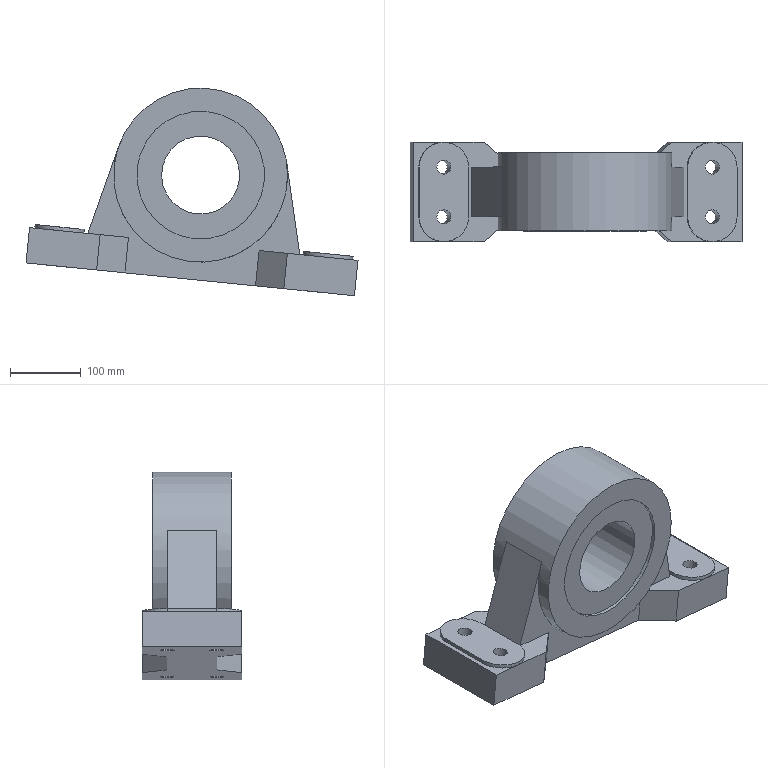Component | NX | BEARING_SEAT1 | 1 solid | 41 faces | volume 6706322 mm3 | plane 29 | cylinder 12 | commonest cylinder face diameters 70 x4 20 x4 180 x2 245 x1 110 x1